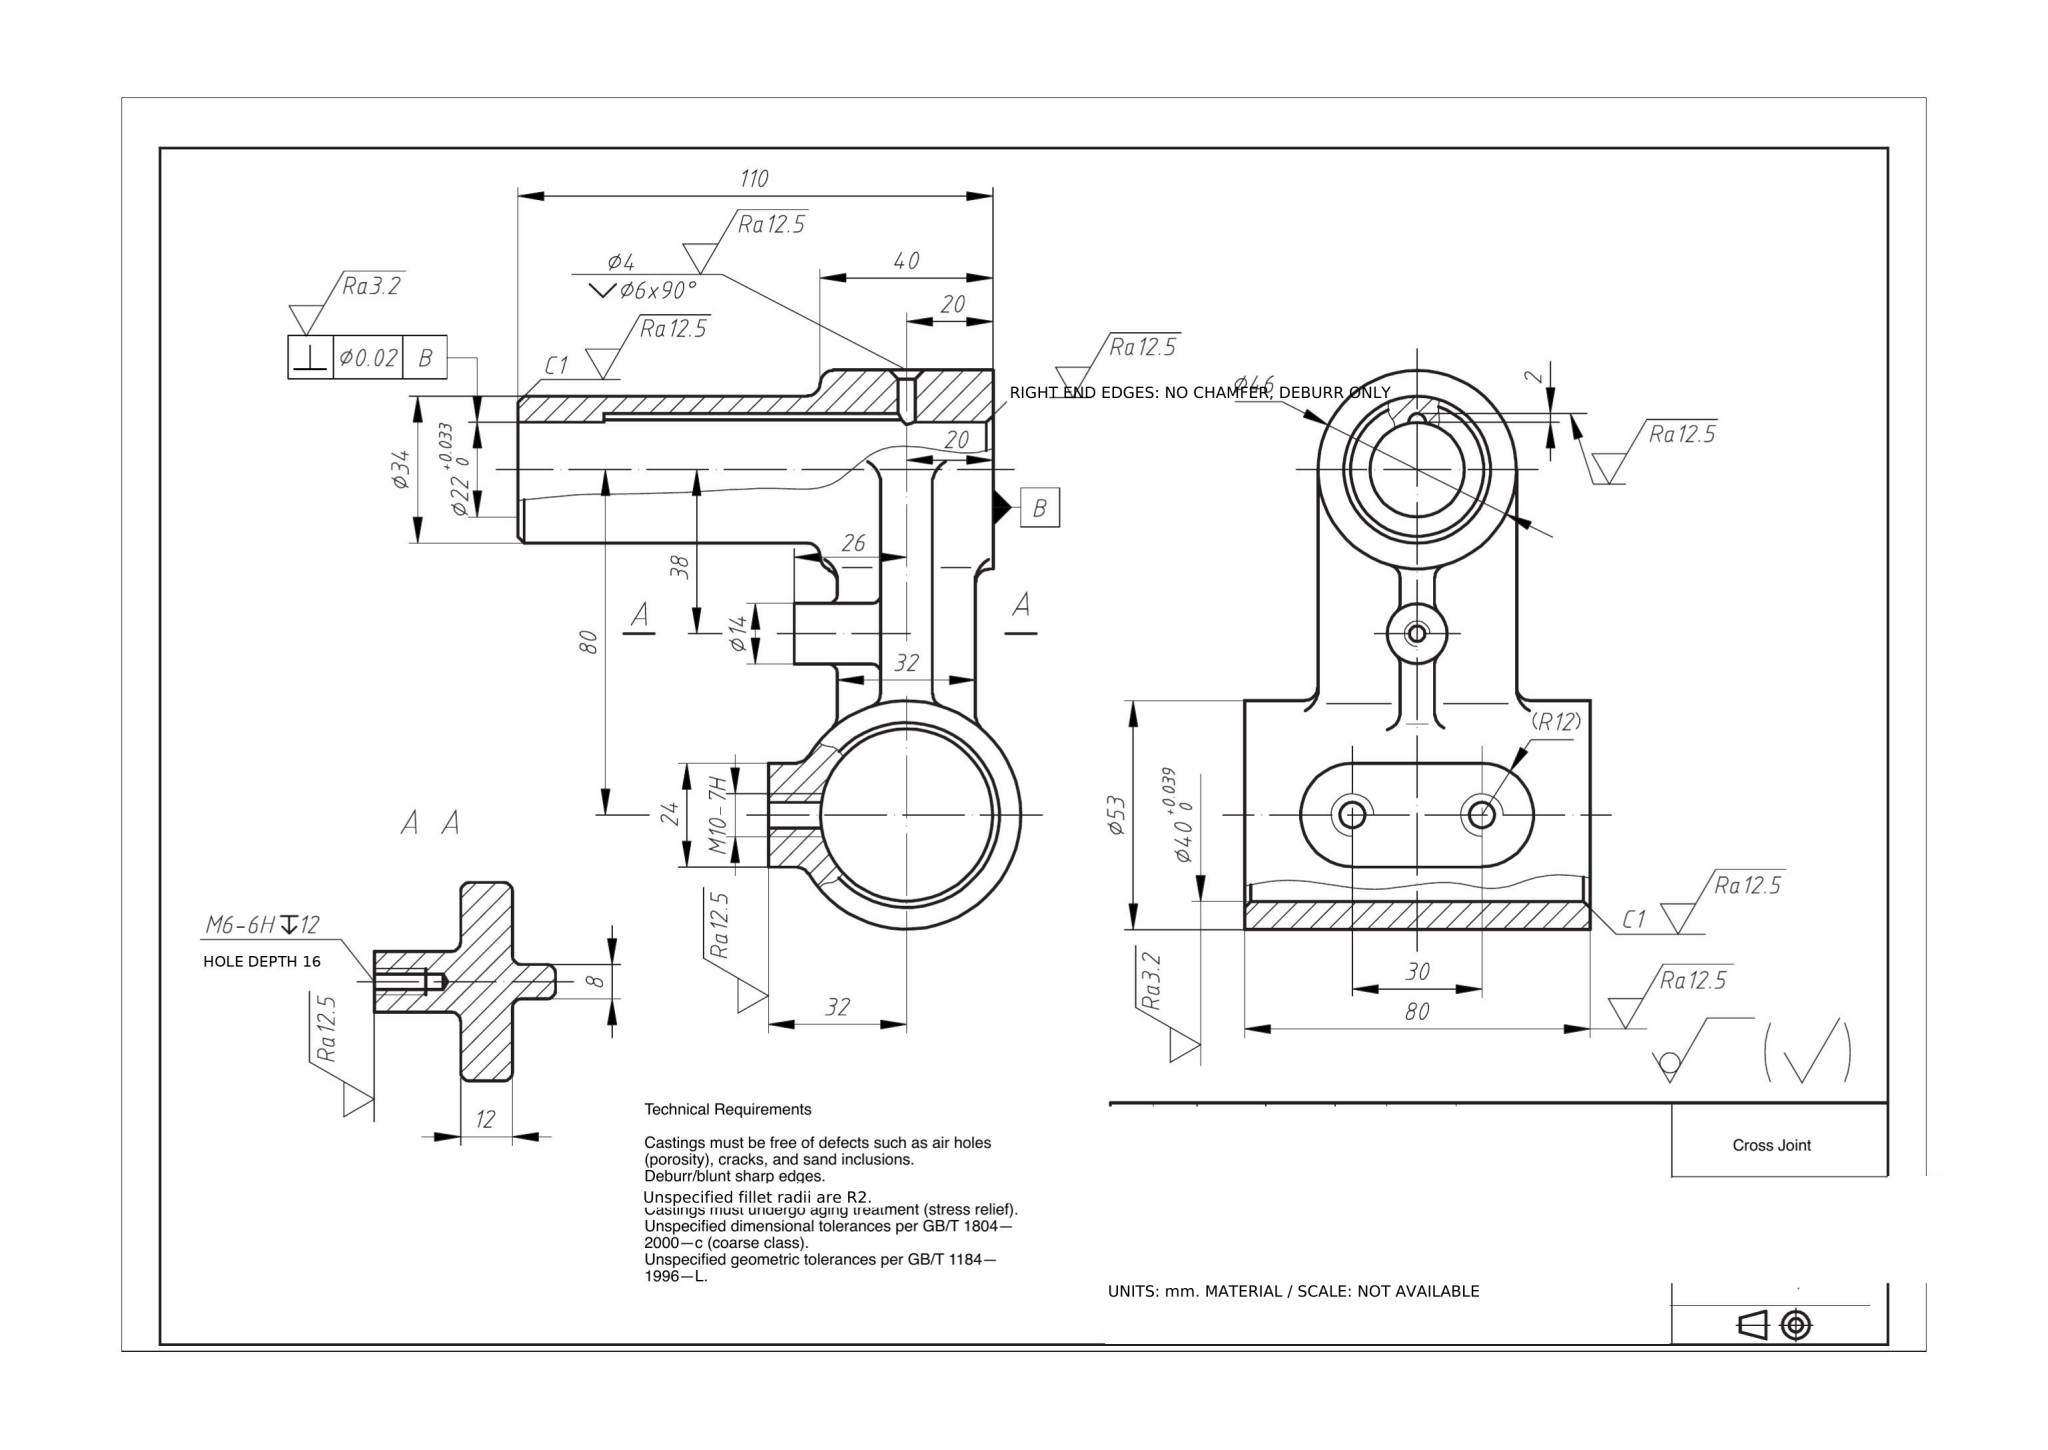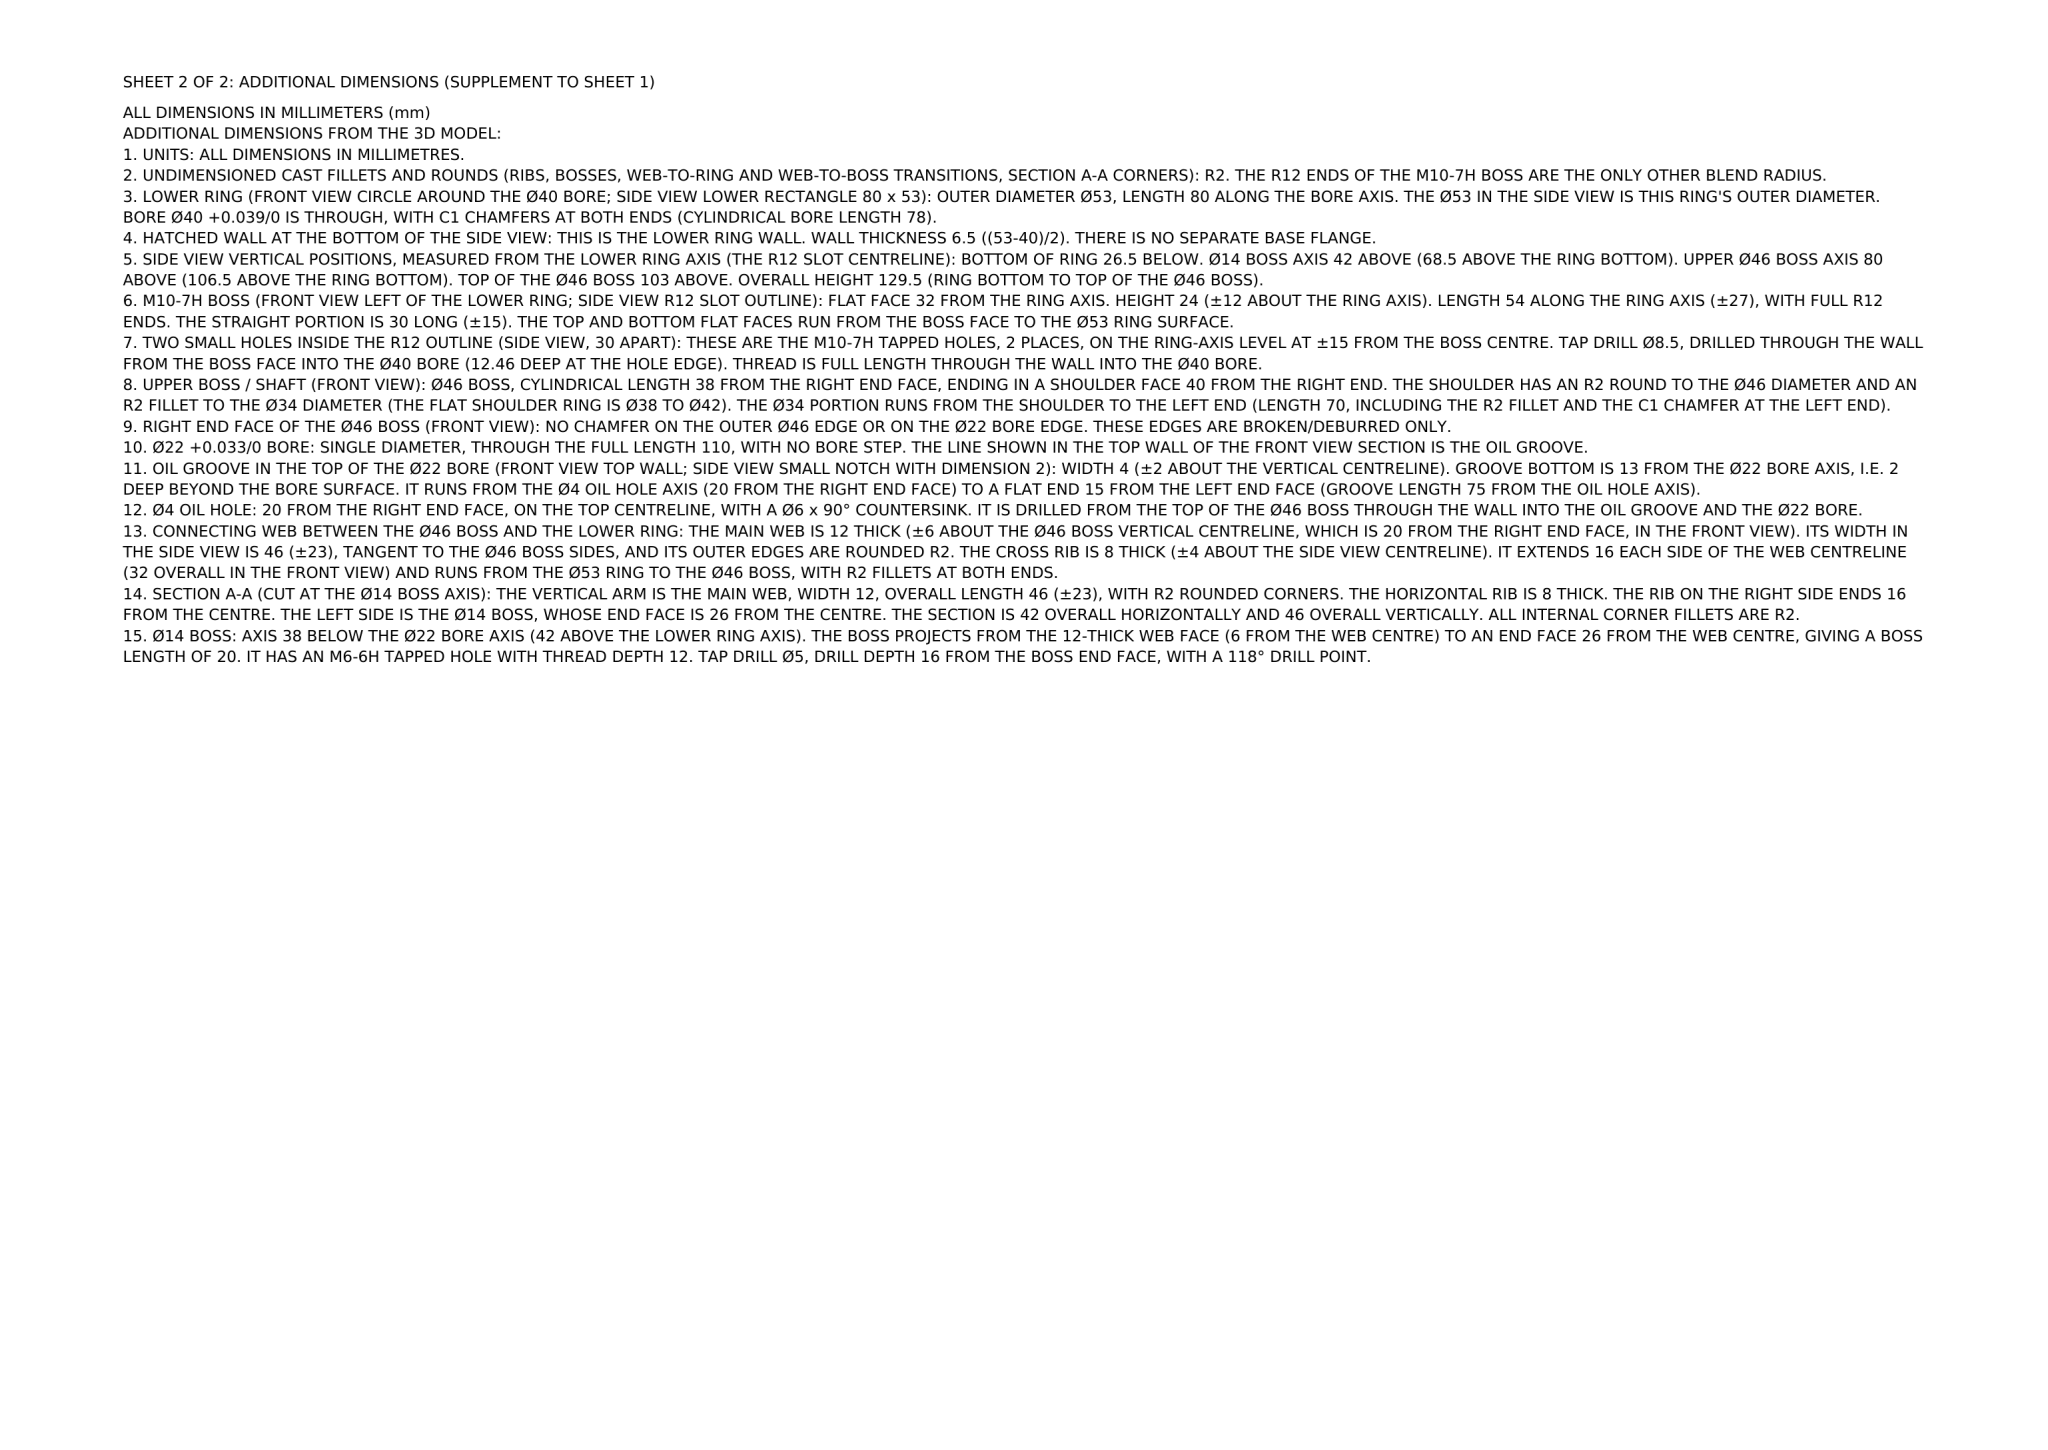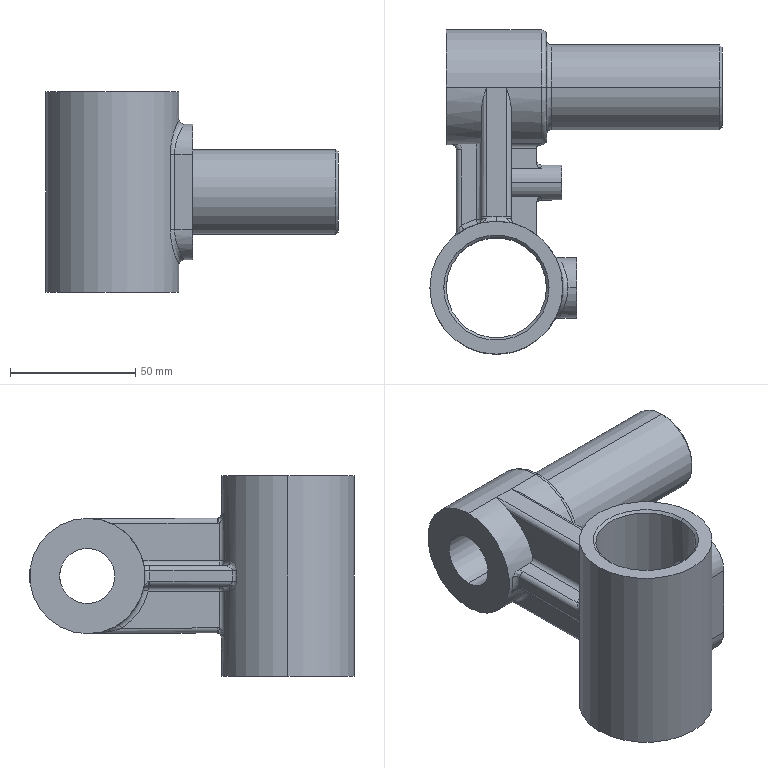Part | NX | mm | 1 solid | 119 faces | box 116.5 x 129.5 x 80 mm | volume 196005 mm3 | cylinder 48 | plane 25 | spline 18 | torus 15 | cone 10 | sphere 3 | commonest cylinder face diameters 4 x26 8.5 x4 24 x3 46 x3 22 x2 5 x2 40 x2 14 x2